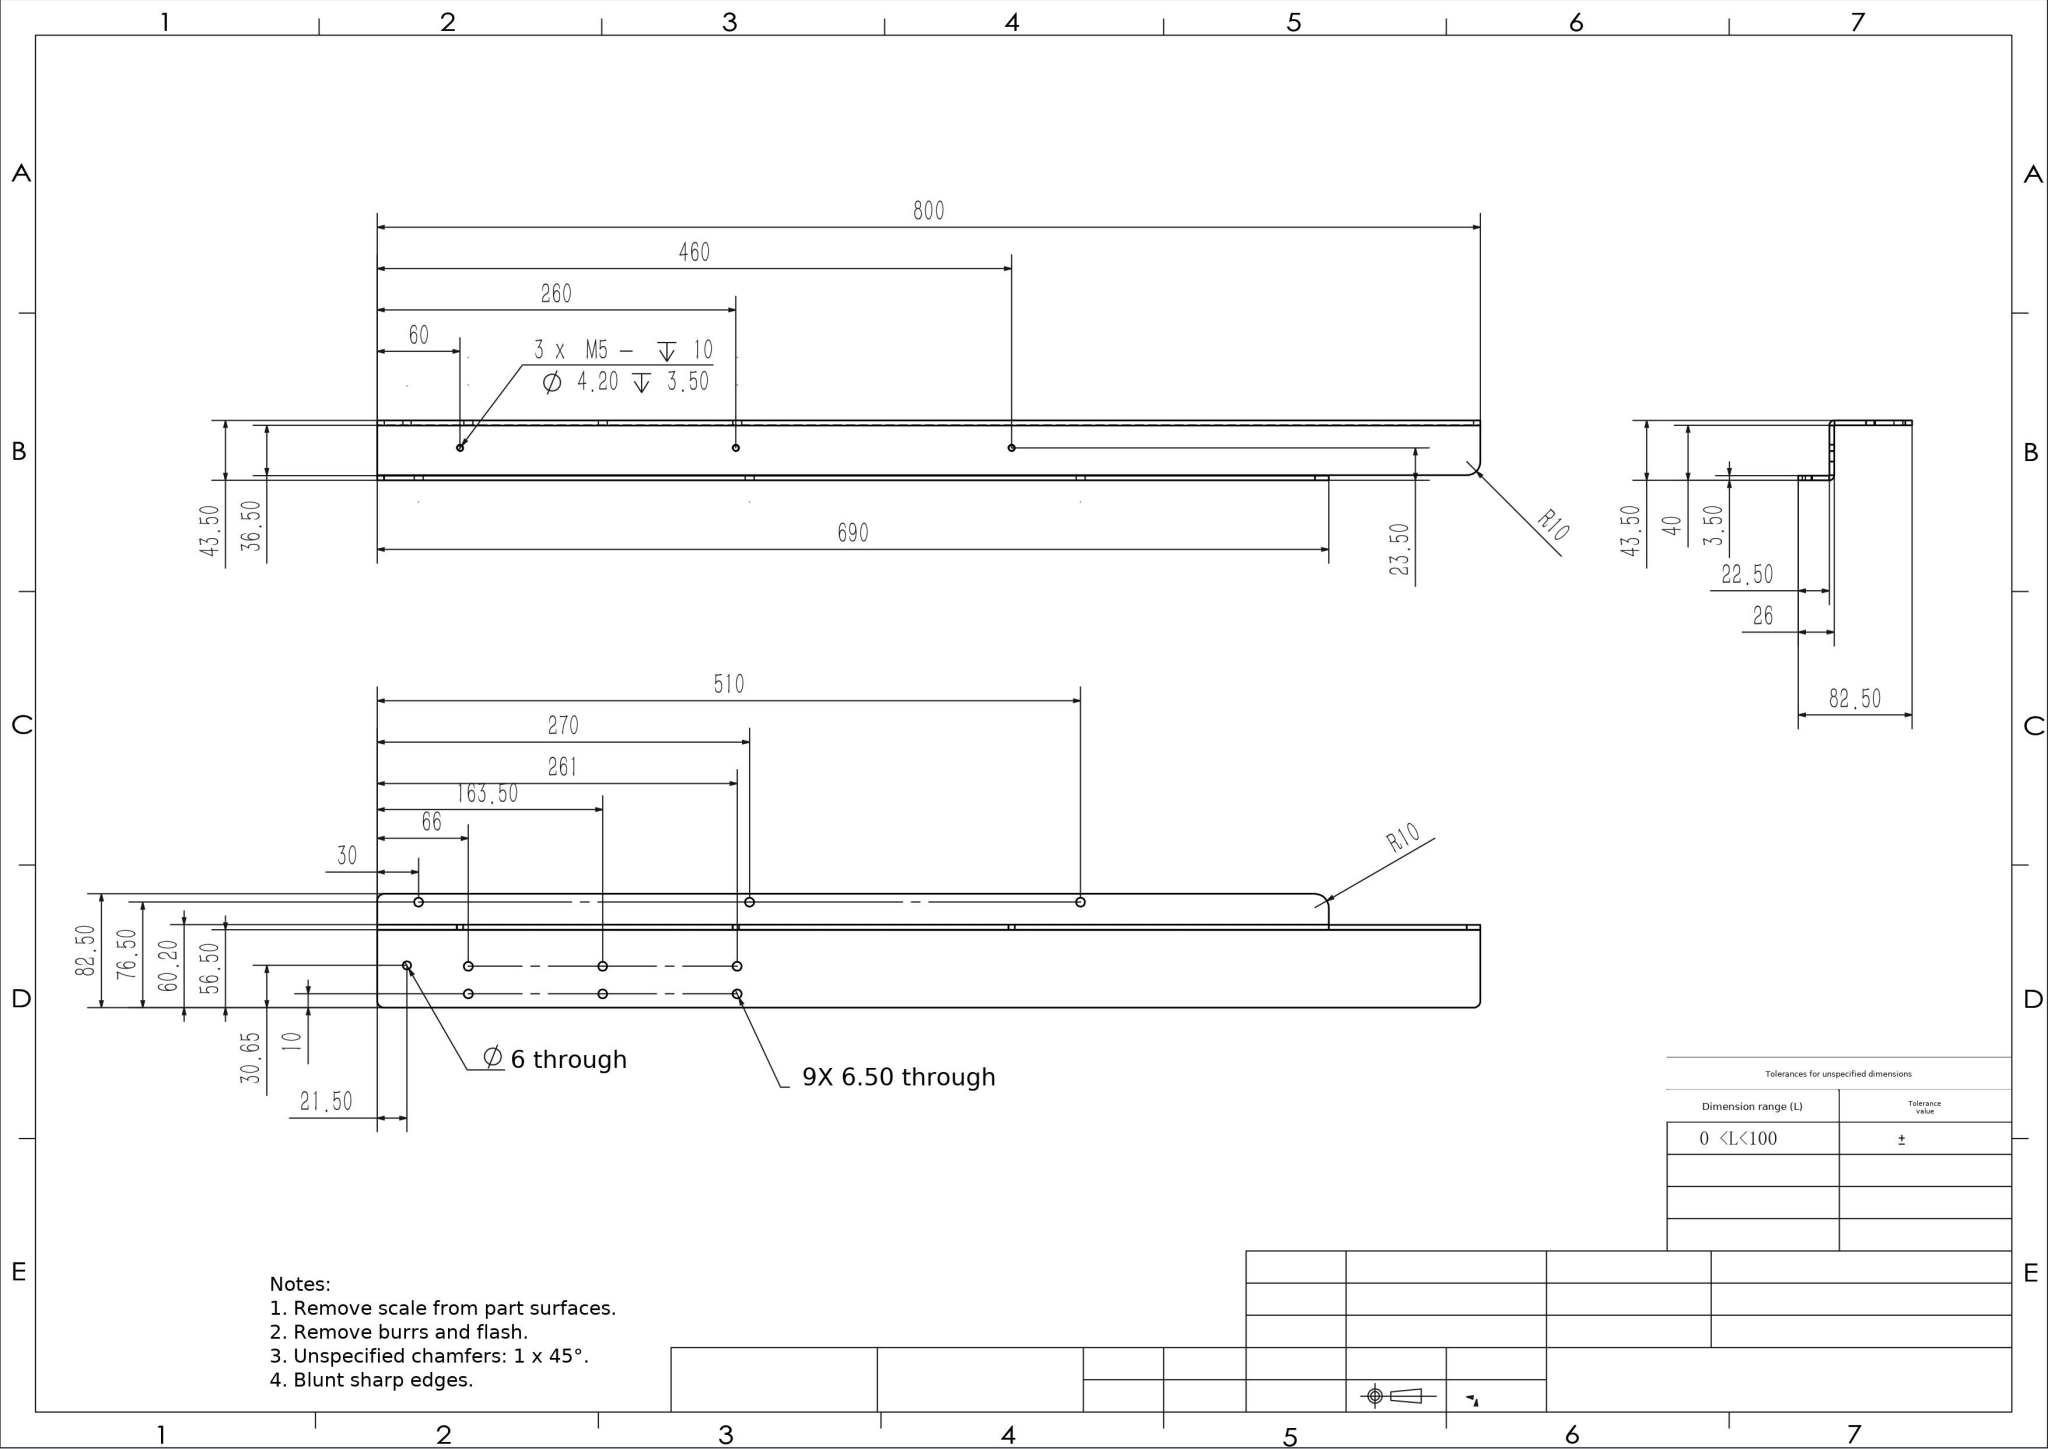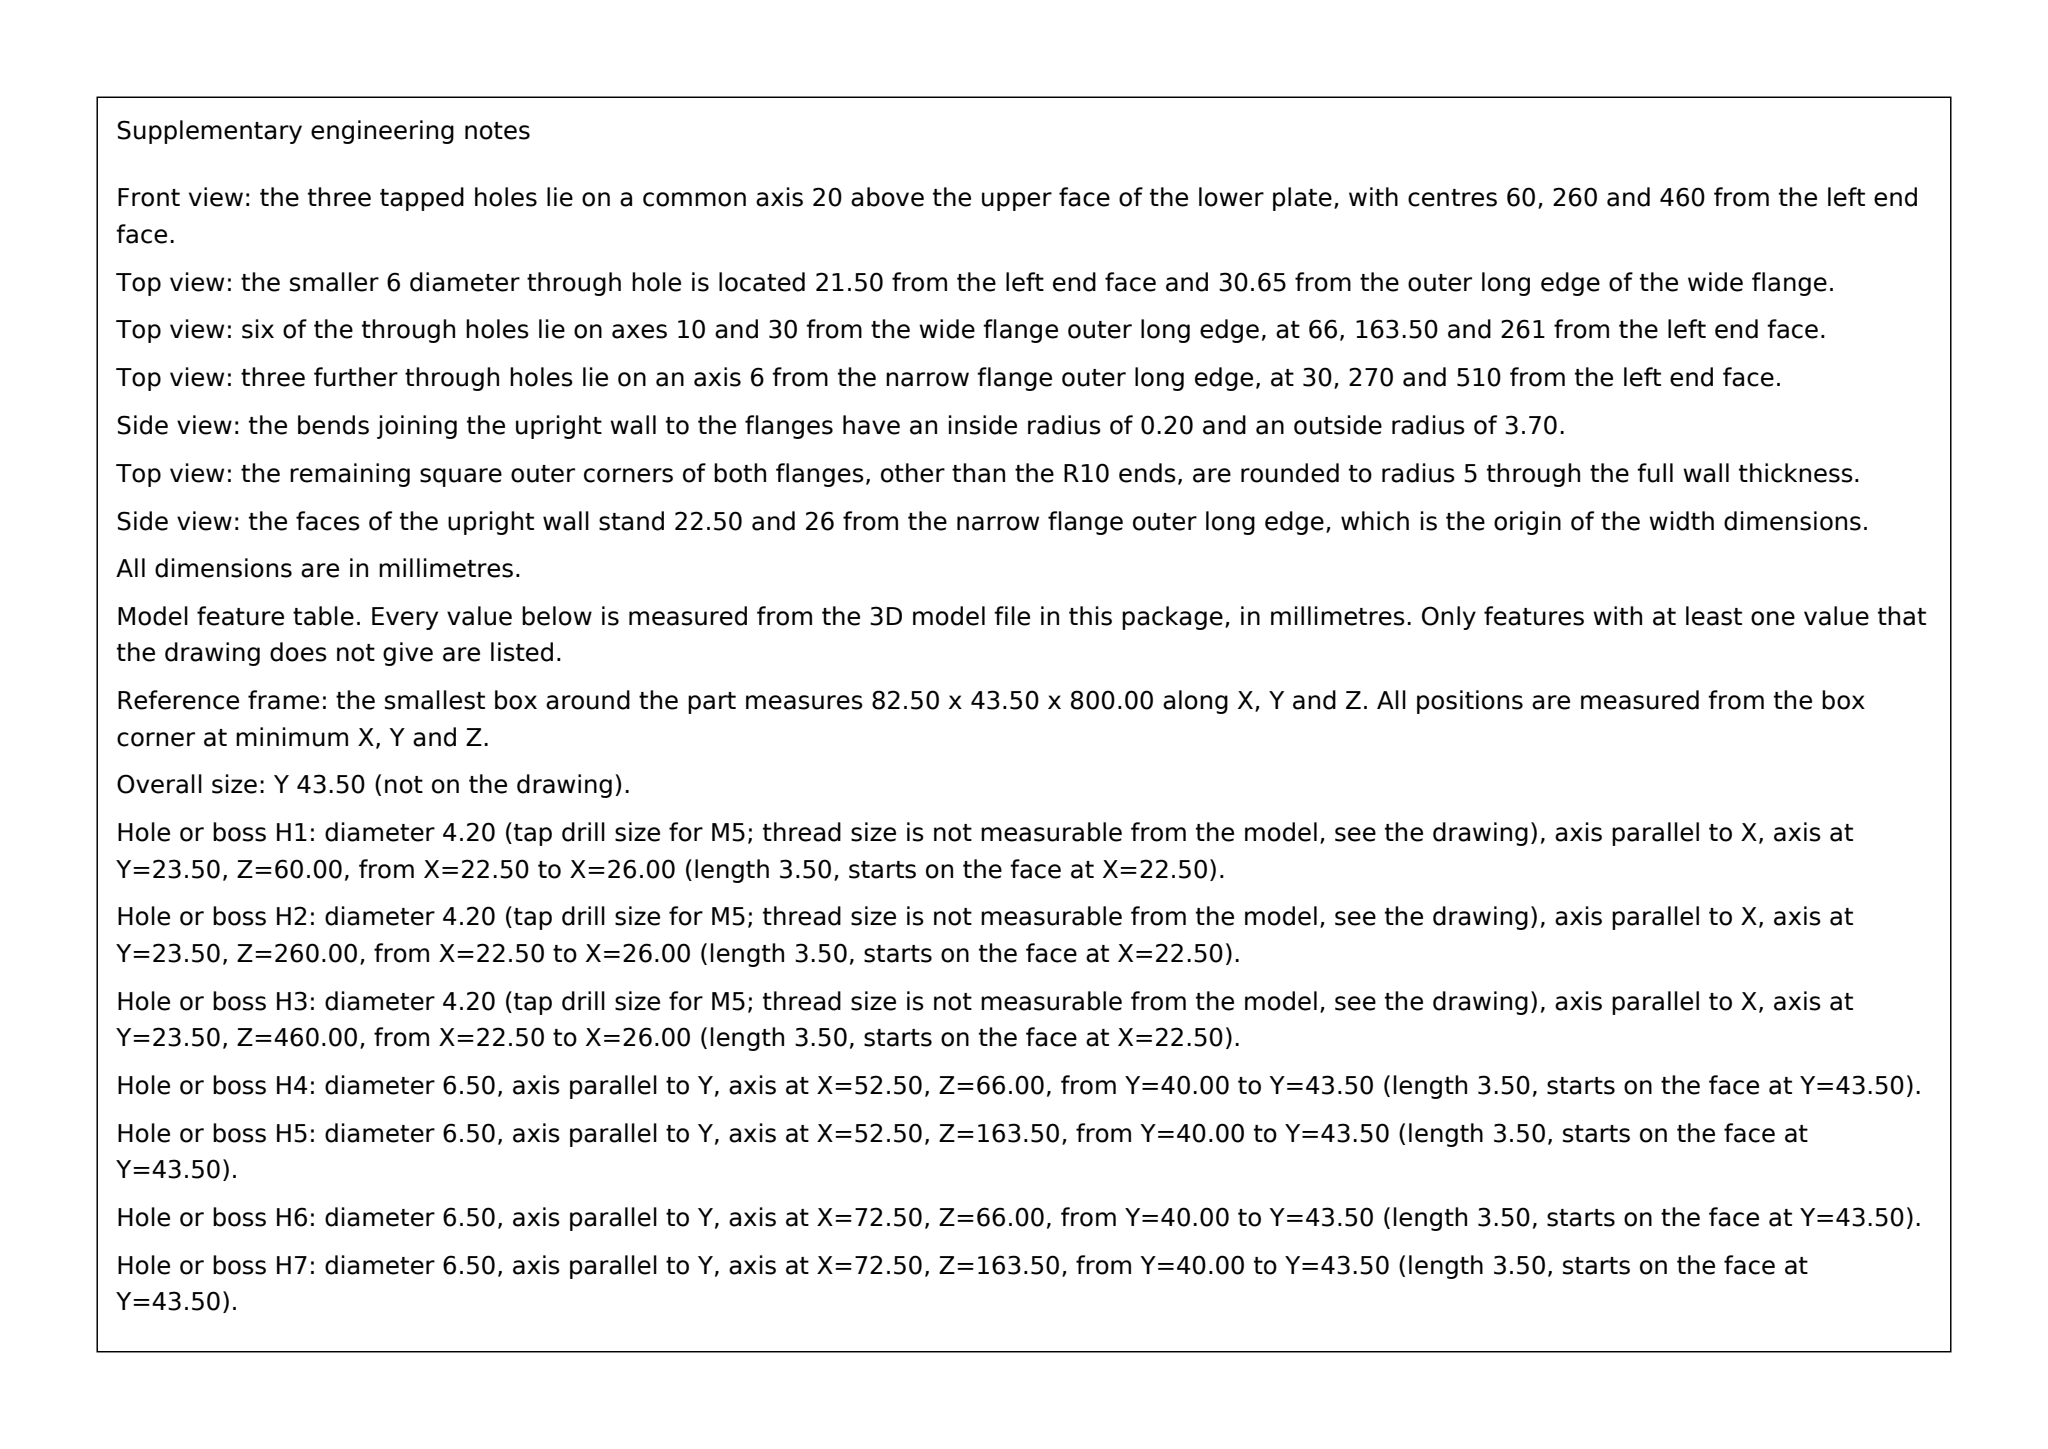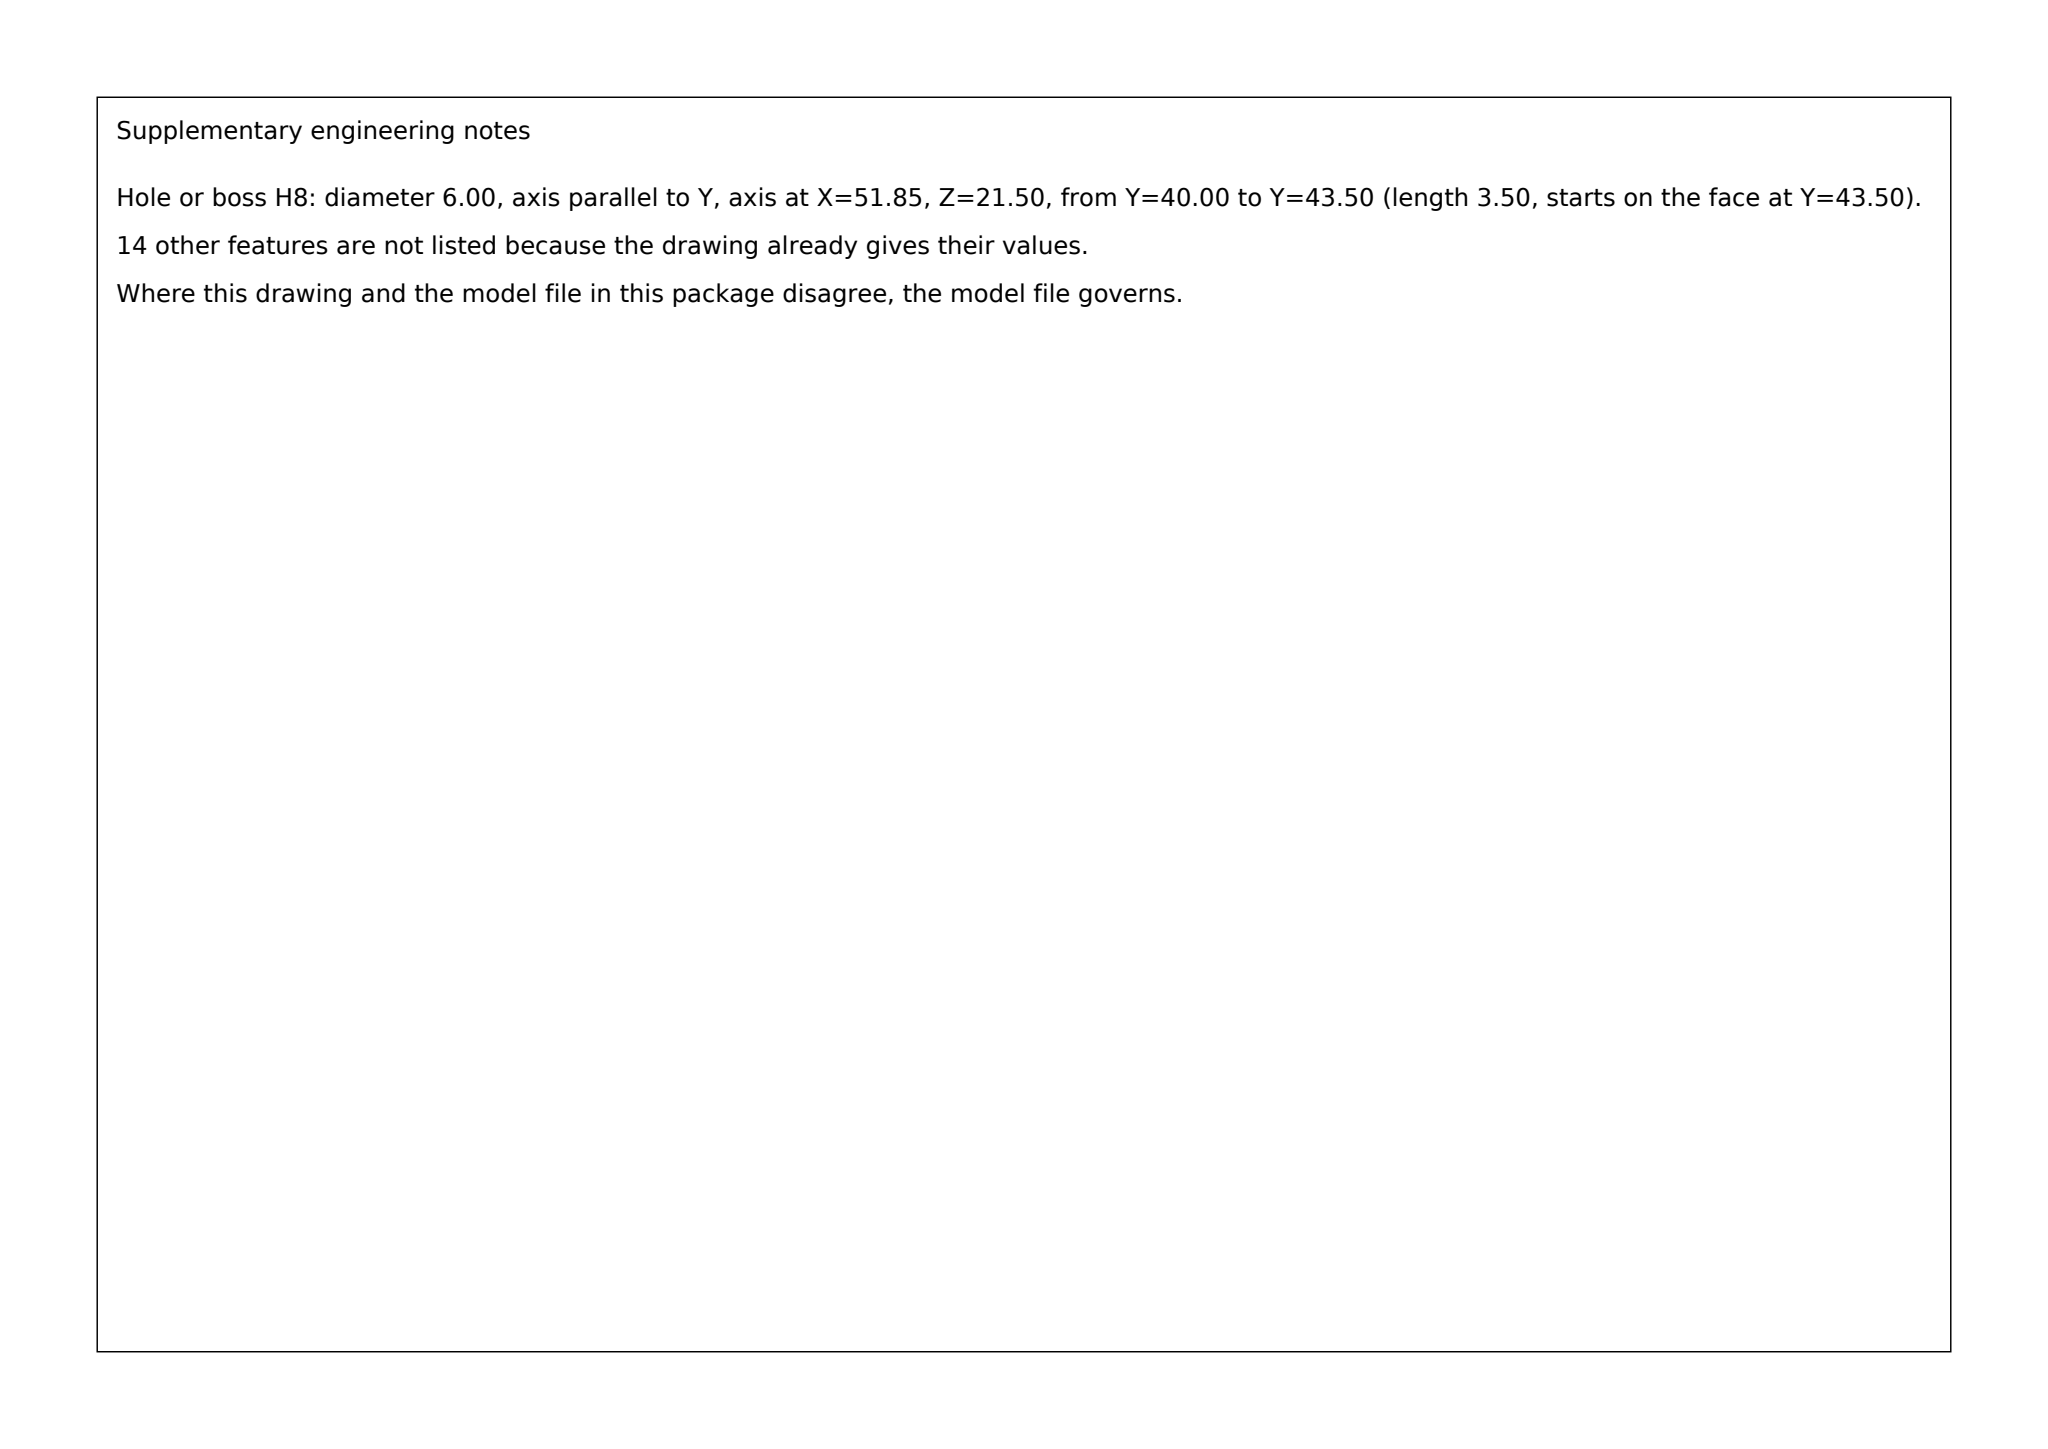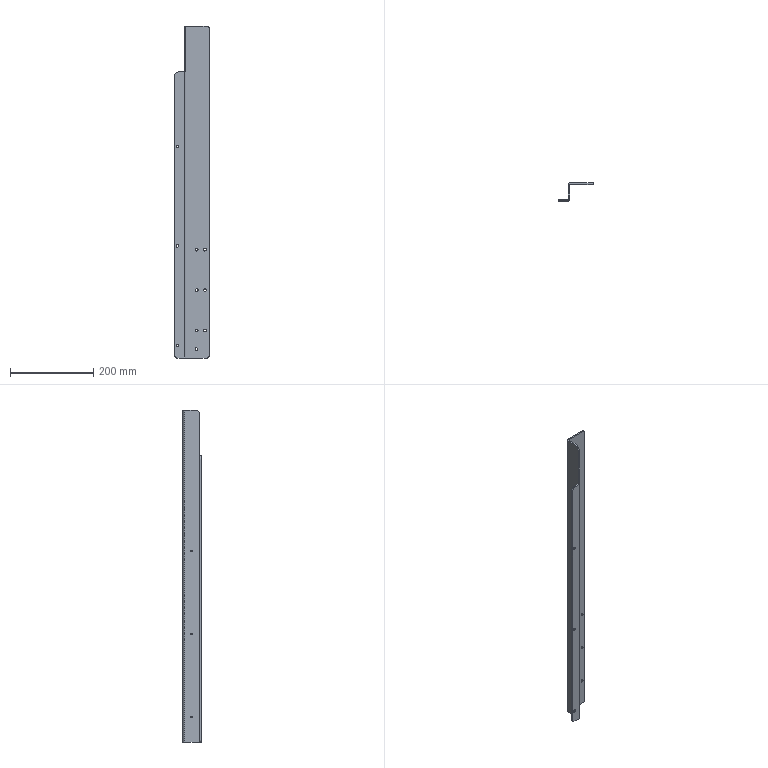Part | SolidWorks | mm | 1 solid | 54 faces | box 82.5 x 43.5 x 800 mm | volume 327052 mm3 | cylinder 35 | plane 19 | commonest cylinder face diameters 6.5 x18 4.2 x6 10 x3 6 x2 0.4 x2 7.4 x2 20 x2